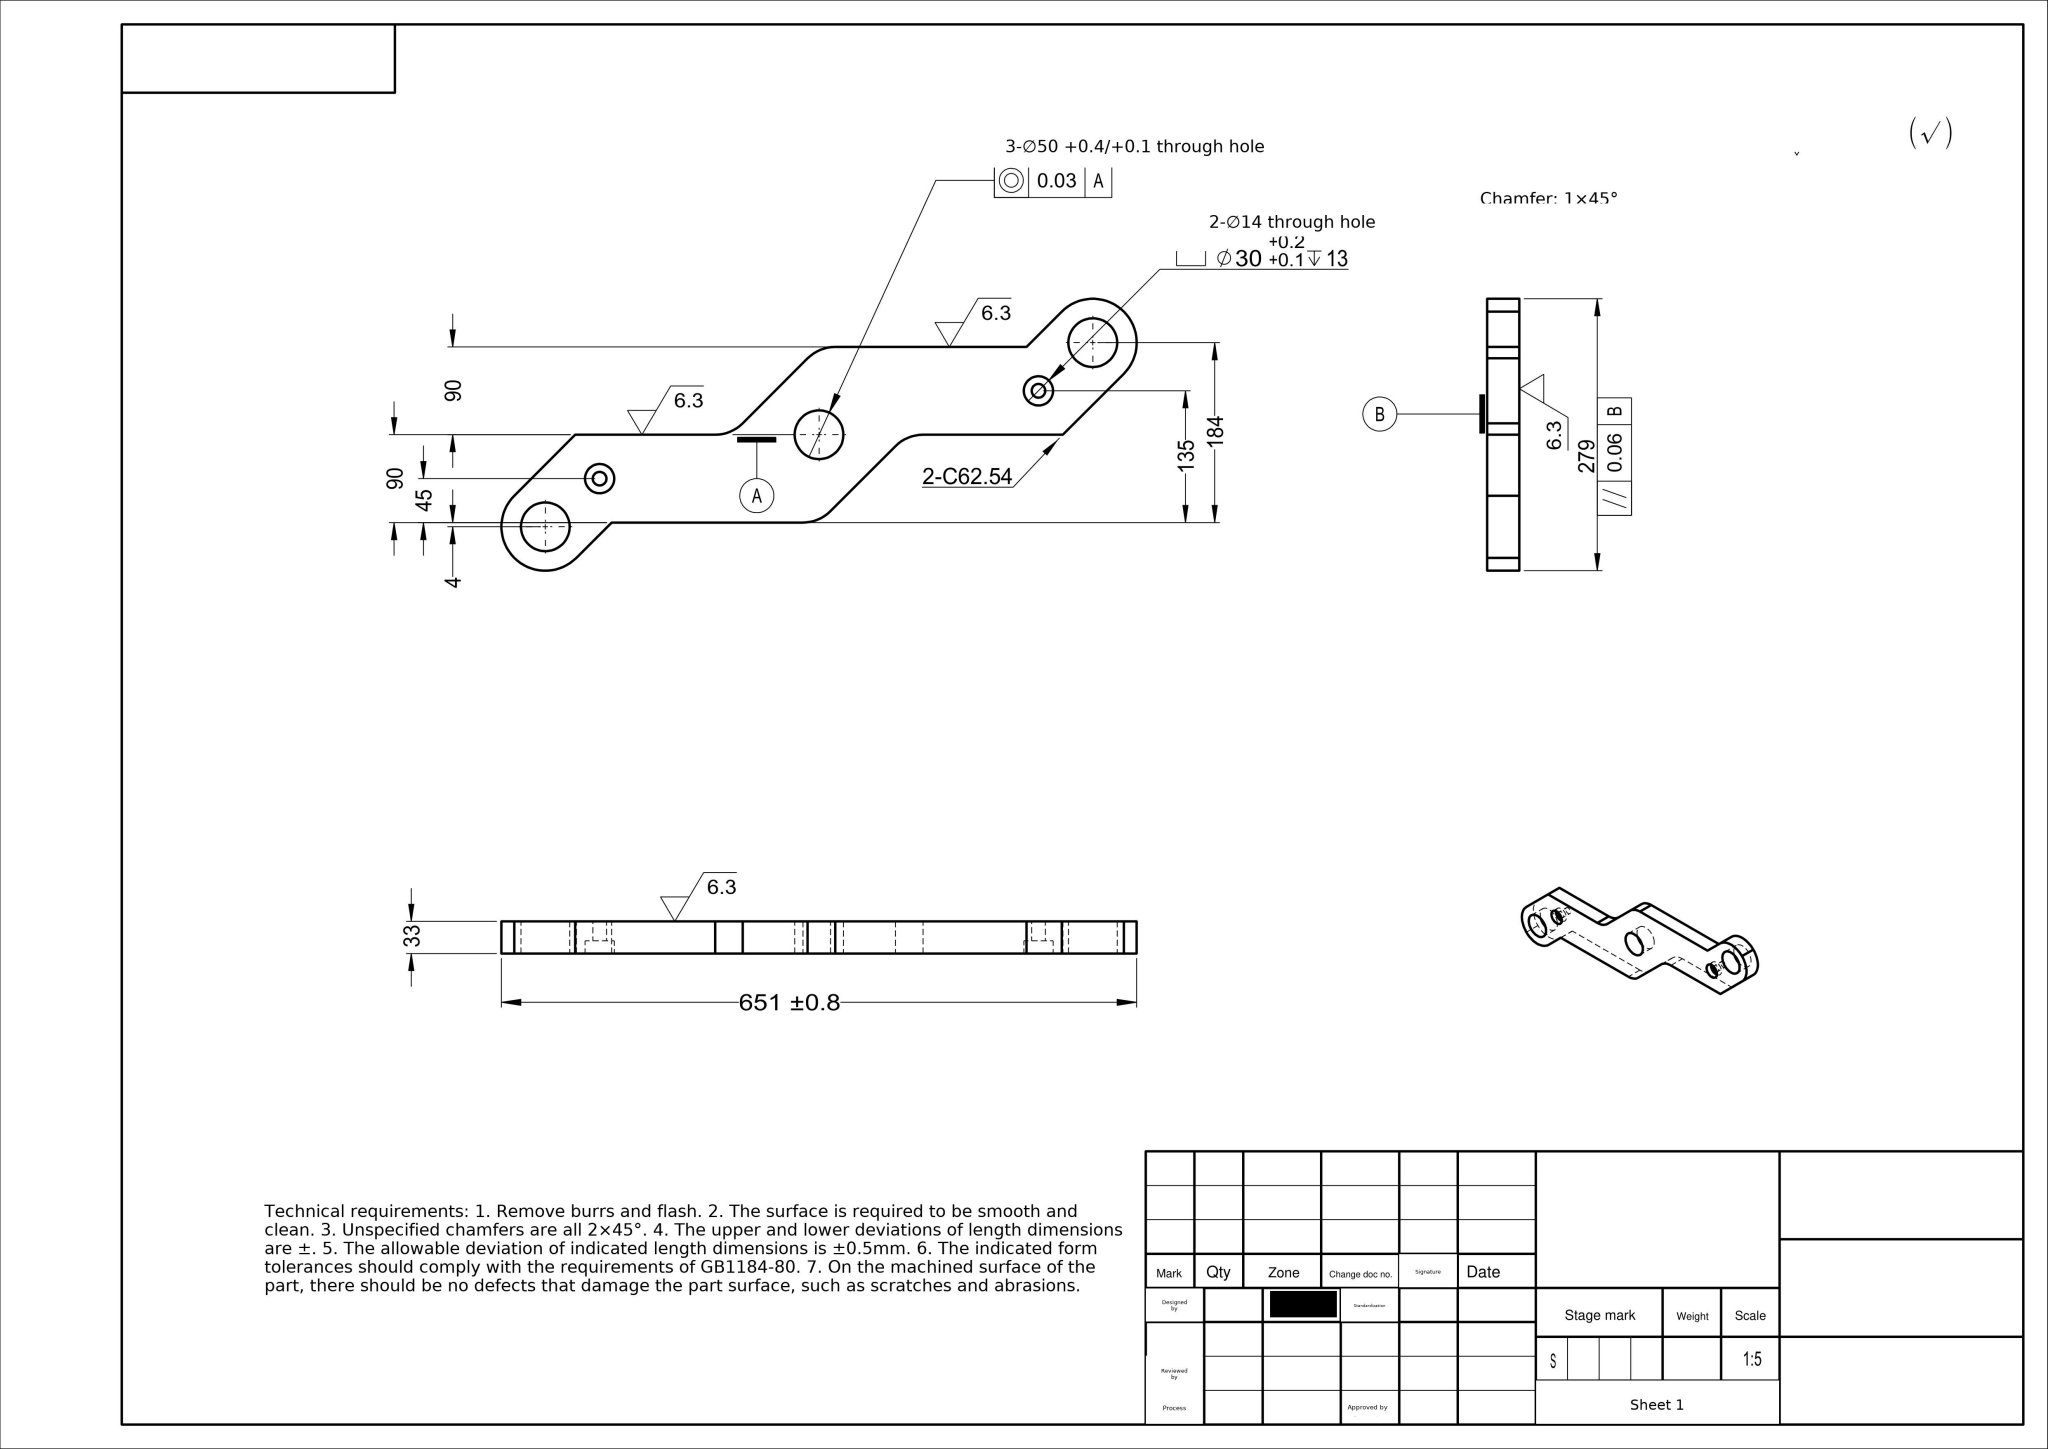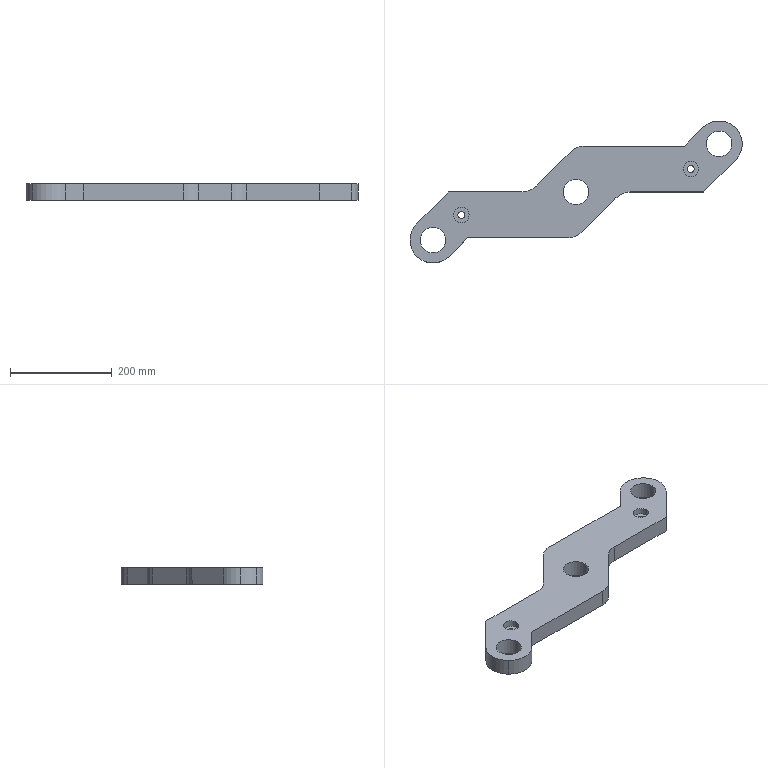Part | SolidWorks | mm | 1 solid | 37 faces | box 651.44 x 278.72 x 33 mm | volume 2047244 mm3 | cylinder 23 | plane 14 | commonest cylinder face diameters 50 x6 90 x5 30 x4 14 x4 80 x4